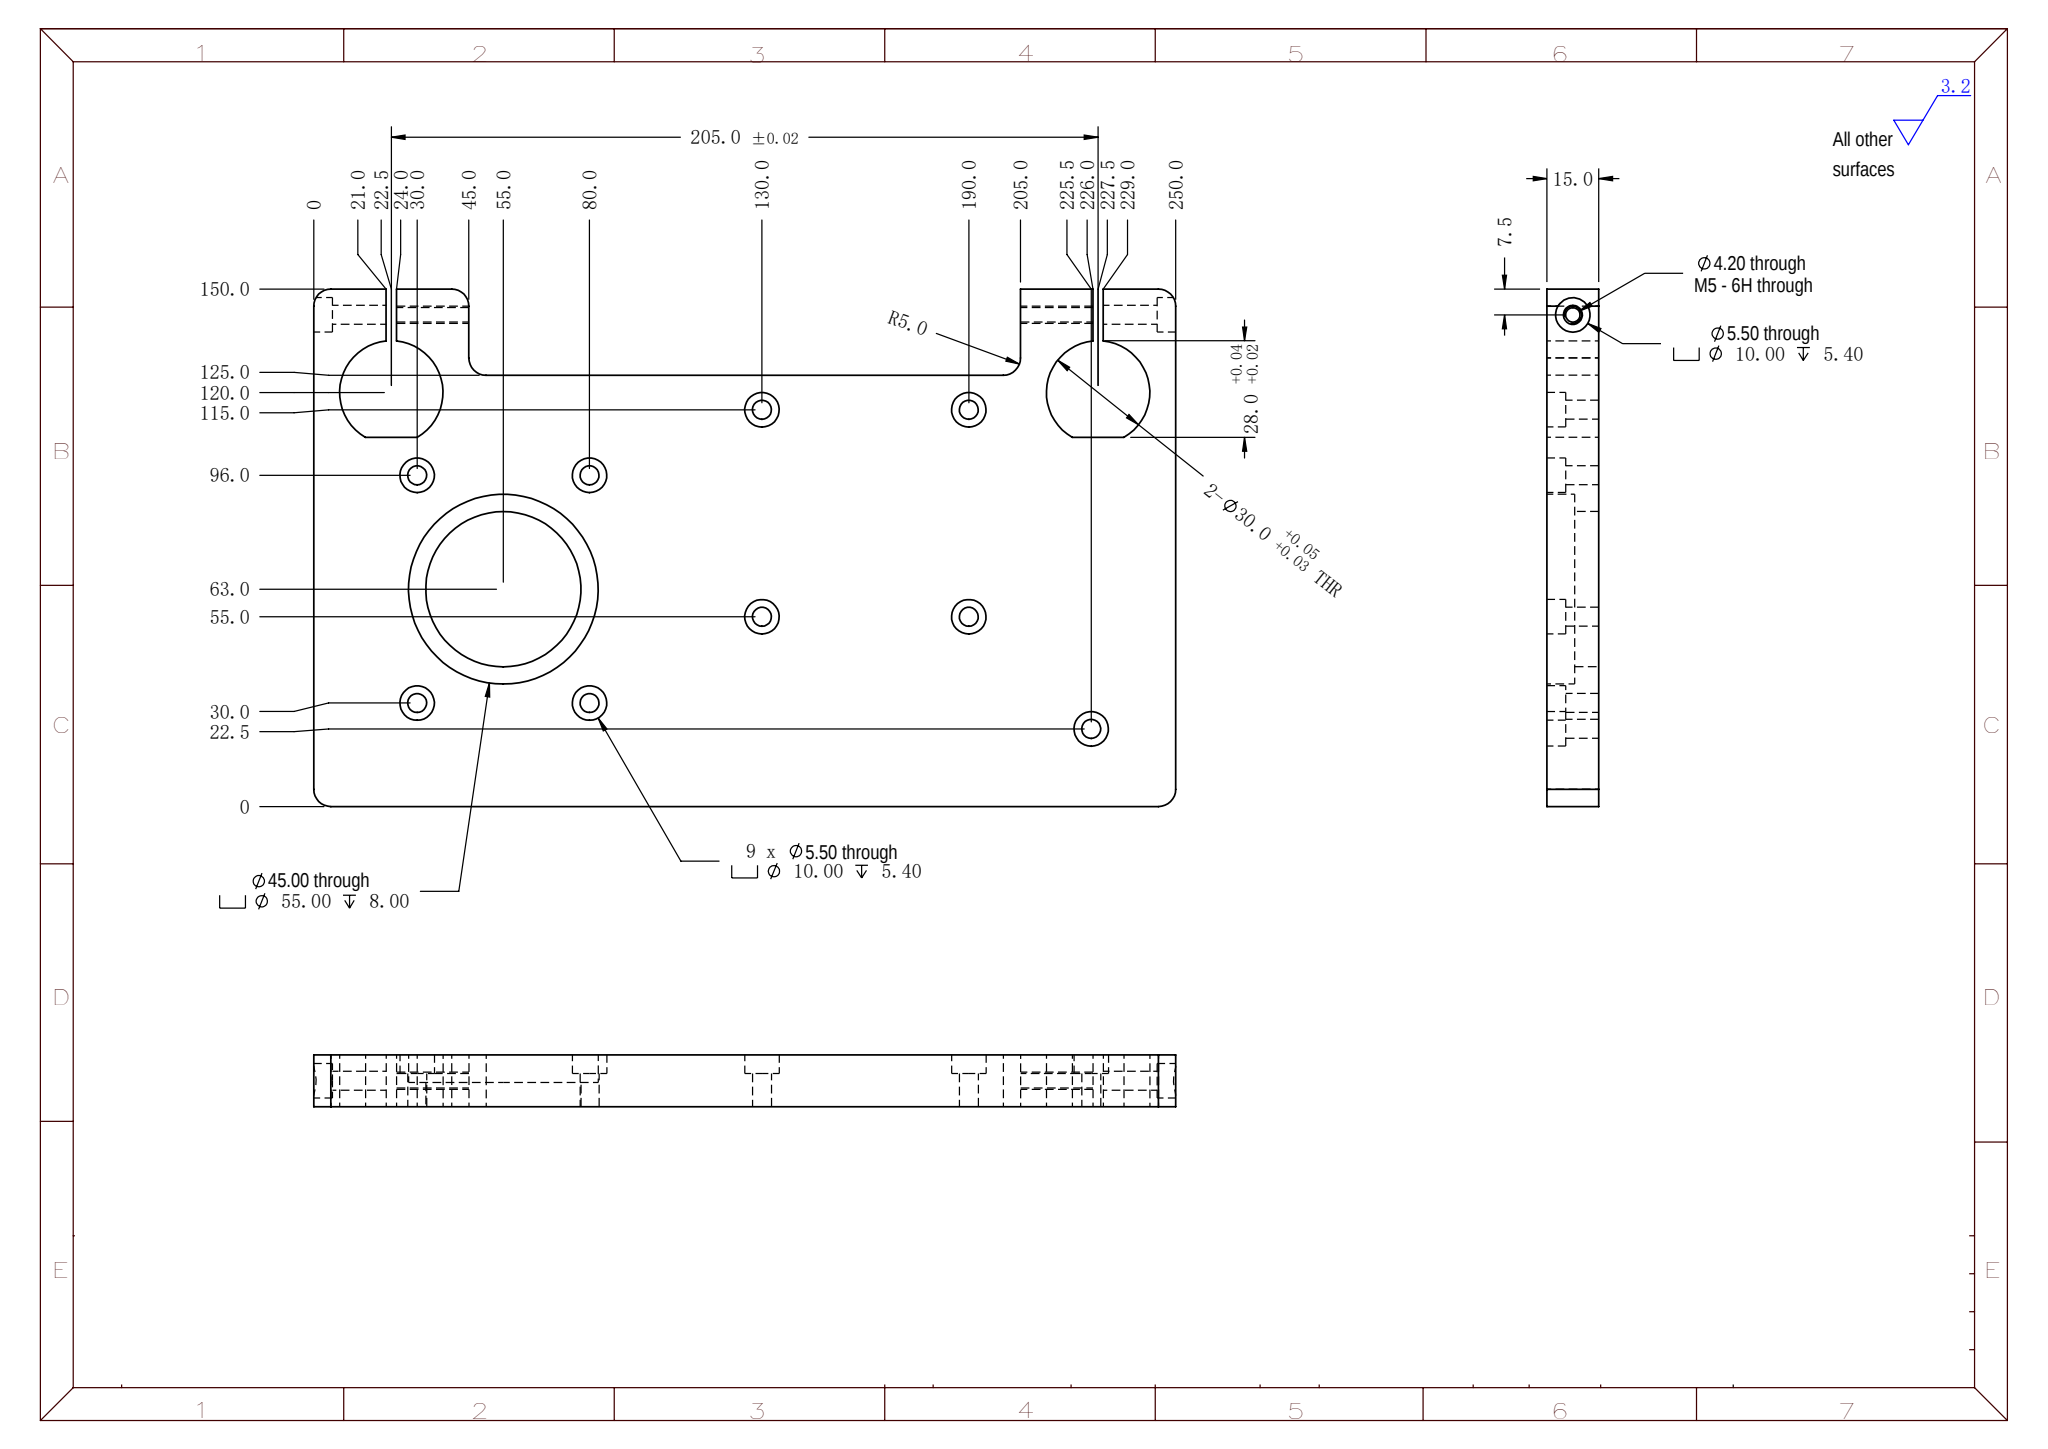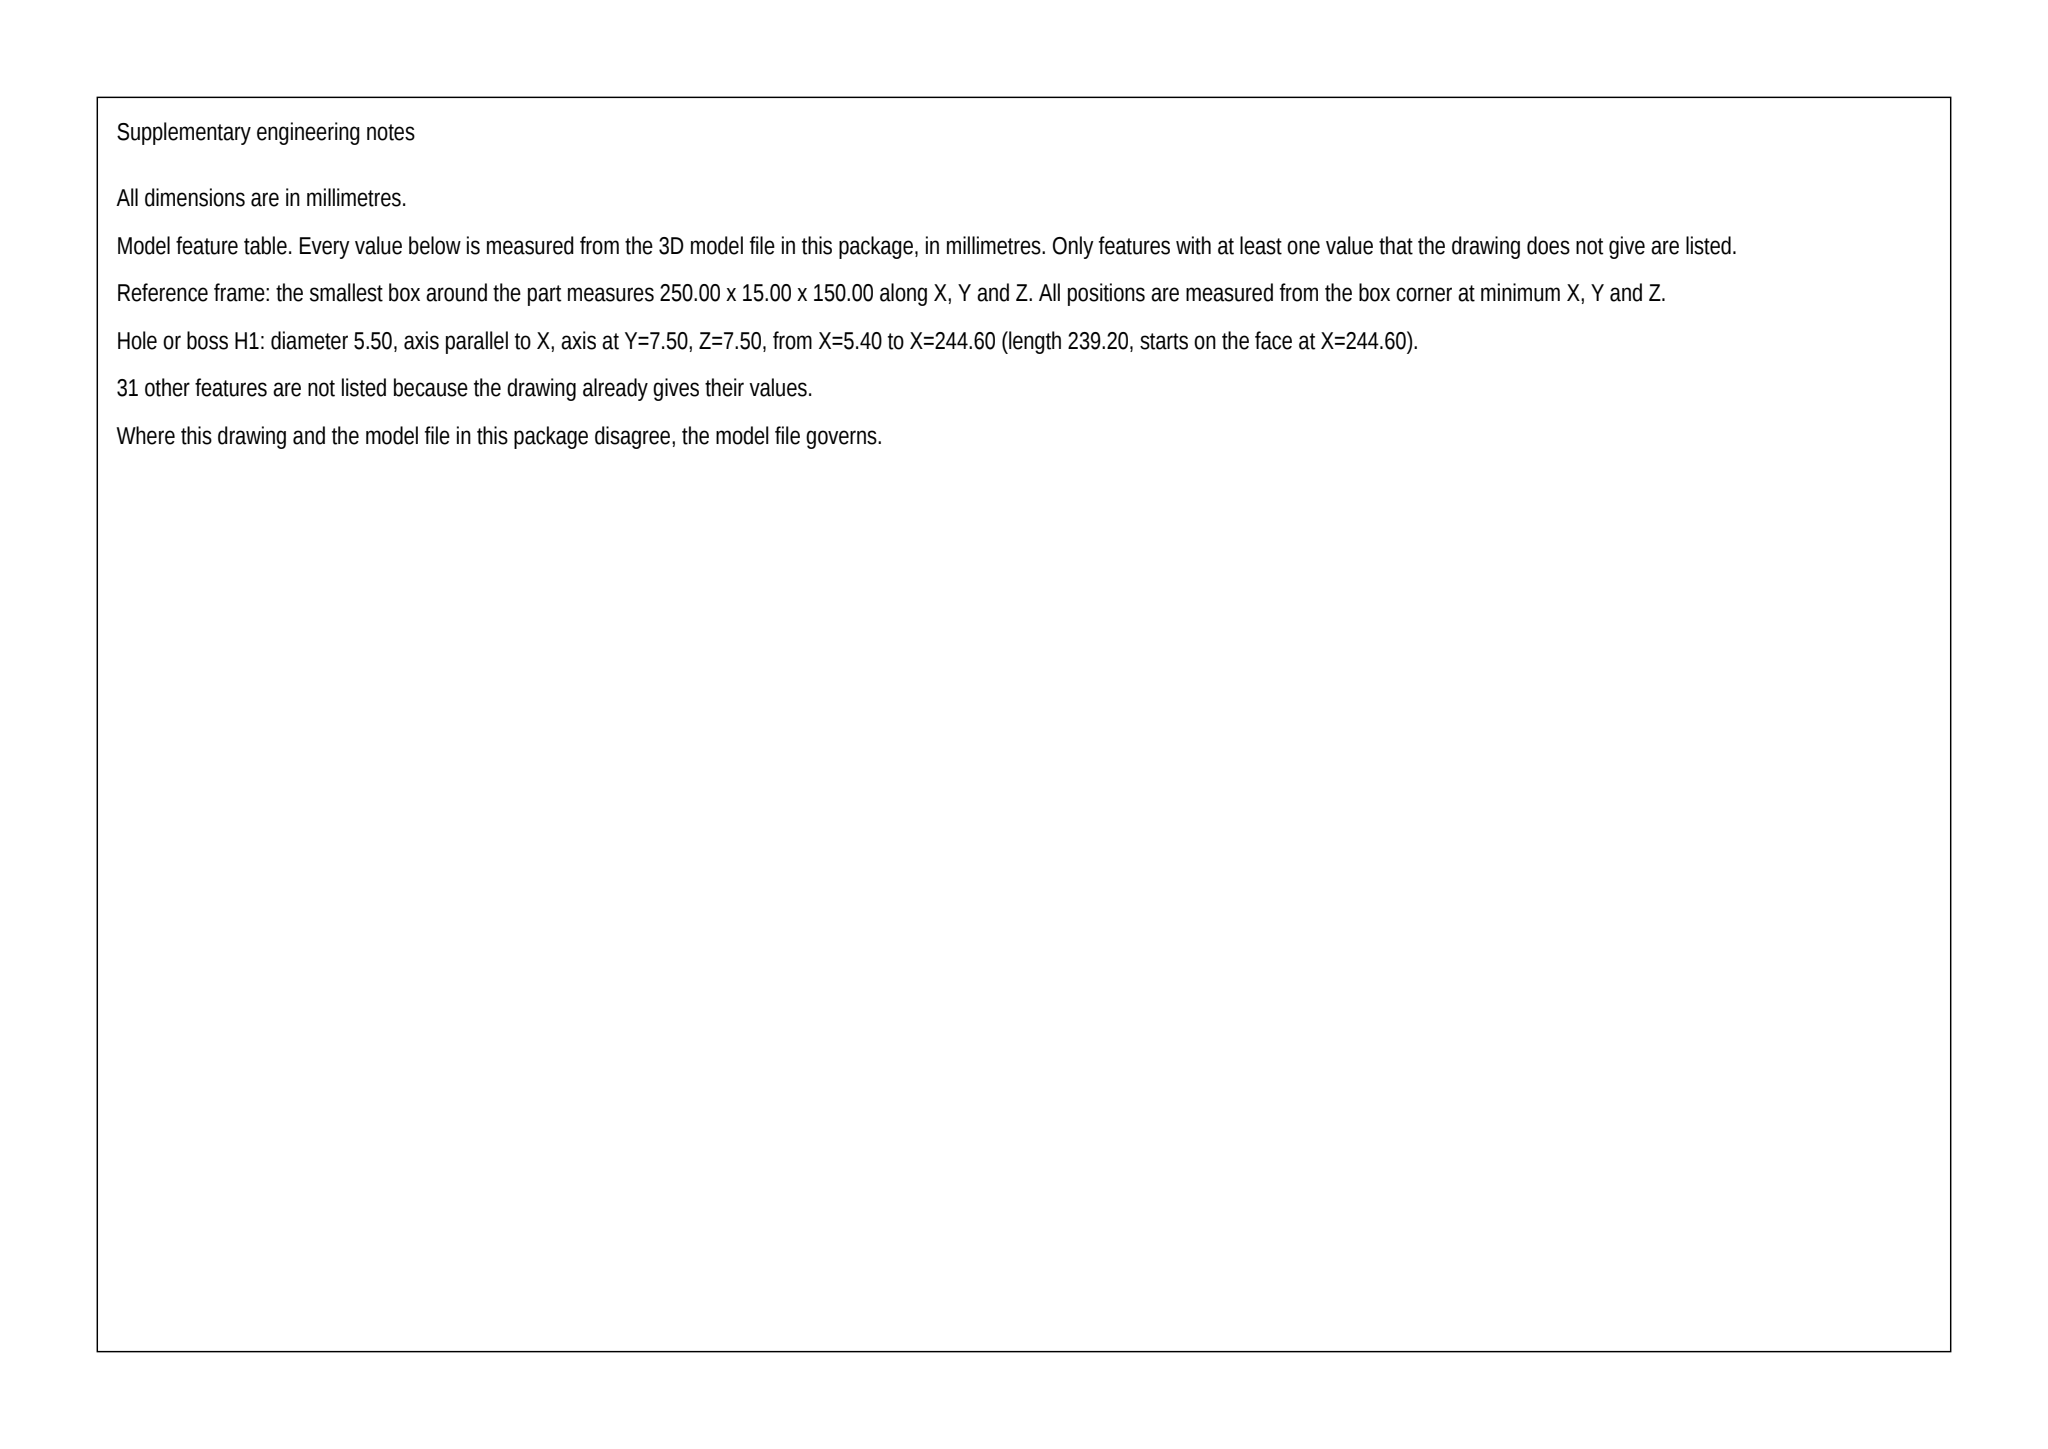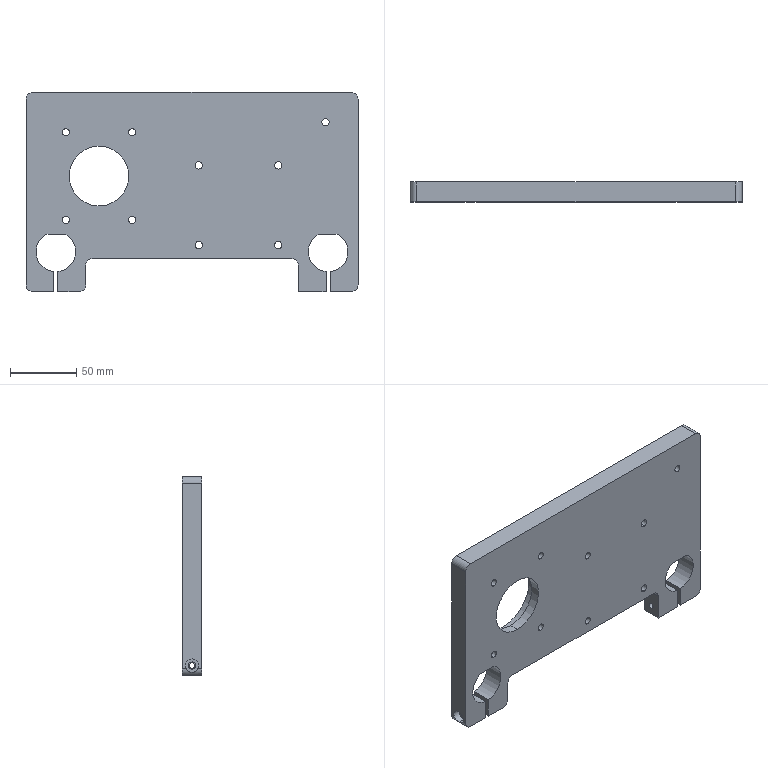Part | SolidWorks | mm | 1 solid | 93 faces | box 250 x 15 x 150 mm | volume 442132 mm3 | cylinder 63 | plane 30 | commonest cylinder face diameters 10 x29 5.5 x22 4.2 x4 30 x4 55 x2 45 x2